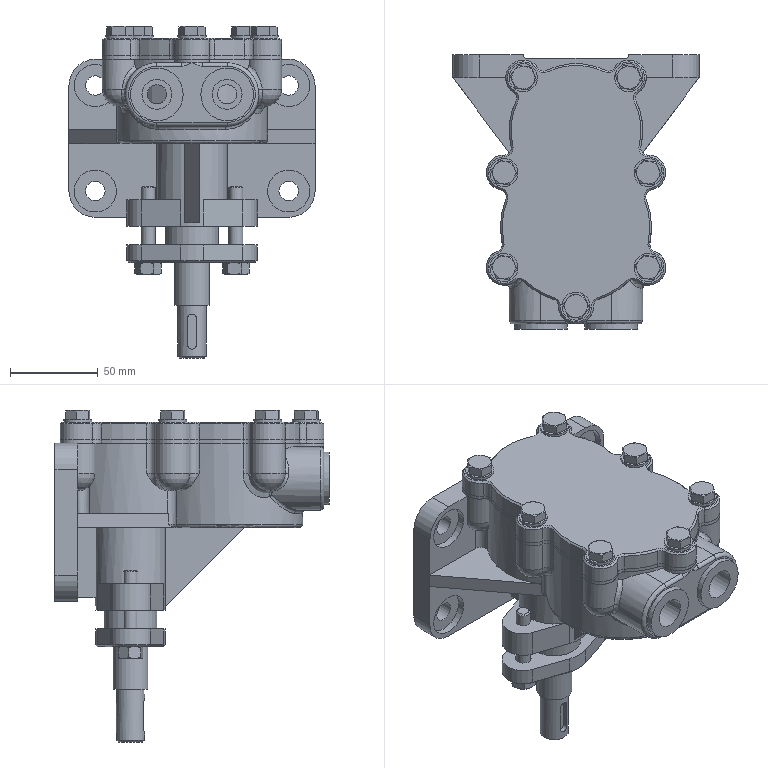Assembly | NX | mm | 27 component files | 32 solids | 522 faces | box 140 x 156 x 188.9 mm | volume 814585 mm3 | cylinder 197 | plane 188 | cone 81 | other 21 | torus 17 | spline 12 | sphere 6 | commonest cylinder face diameters 8 x58 20 x26 10 x14 86 x11 16 x9 30 x9 25 x9 76 x8
Bill of materials:
unnamed part 1 | 2 |  | Hexagonal nut-like prism with a central plain cylindrical through-bore and chamfered corners on both faces.
unnamed part 2 | 2 |  | Plain solid cylindrical rod or pin with small chamfers at both ends.
unnamed part 3 | 1 |  | Thin flat gasket-like plate with a figure-eight opening made of two overlapping circles, and seven rounded perimeter lugs, each with a through-hole.
unnamed part 4 | 1 |  | Solid flat plate with a lobed outline formed by two merged circles, and seven rounded lugs with through-holes around the edge. It looks like a cover plate.
unnamed part 5 | 7 |  | Hex-head bolt-like part: a hexagonal head with a chamfered top, on a plain cylindrical shank with a chamfered tip.
unnamed part 6 | 1 |  | Stepped cylindrical shaft with a thin disk-shaped collar near one end. A smaller pin sits above the collar, offset from the main axis. The opposite end steps down to a smaller diameter with a slot or flat.
unnamed part 7 | 1 |  | Thin-walled cylindrical tube or sleeve with plain ends and a small axial groove along the bore.
unnamed part 8 | 1 |  | Short solid cylinder with one radial through-hole across its diameter.
unnamed part 9 | 1 |  | Thick annular ring or bushing with a central through-bore and large chamfers on the outer edges at both ends.
unnamed part 10 | 7 |  | Complex housing-like body. It has a double-bore cavity shaped like a figure eight, surrounded by a flange with seven bolt holes, and is joined at right angles to a rectangular mounting plate with four corner holes. It also has cylindrical bosses or ports and a triangular stiffening rib.
unnamed part 11 | 1 |  | Solid cylindrical pin with chamfered ends, five shallow evenly spaced circumferential grooves along most of its length, and a radial through-hole near one end.
unnamed part 12 | 1 |  | Flat circular washer-like ring with a plain central hole and uniform thickness.
unnamed part 13 | 1 |  | Two-hole flanged cylindrical boss: a flat diamond/oval-shaped flange plate with rounded lobes, a through hole in each lobe, and a central raised cylindrical hub with a through bore.
Mates:
1. parallel | 6_disk 1 face | 1_pump_body 1 face
2. concentric | 2_side_cover 1 edge | 5_gasket 1 edge
3. concentric | 2_side_cover 1 edge | 5_gasket 1 edge
4. touch align | 6_disk 1 face | 11_plunger 1 face
5. touch align | 10_crankshaft 1 face | 1_pump_body 1 face
6. touch align | 10_crankshaft 1 face | 11_plunger 1 face
7. touch align | 10_crankshaft 1 face | 1_pump_body 1 face
8. concentric | packing 1 edge | 7_bushing 1
9. touch align | 9_packing_gland 1 face | 1_pump_body 1 face
10. concentric | 4_washer_8 7 edge | 2_side_cover 1 edge
11. concentric | 4_washer_8 5 edge | 2_side_cover 1 edge
12. concentric | 4_washer_8 4 edge | 2_side_cover 1 edge
13. concentric | 4_washer_8 6 edge | 2_side_cover 1 edge
14. concentric | 4_washer_8 1 edge | 2_side_cover 1 edge
15. concentric | 4_washer_8 2 edge | 2_side_cover 1 edge
16. concentric | 4_washer_8 3 edge | 2_side_cover 1 edge
17. concentric | 13_nut 2 | 9_packing_gland 1 edge
18. concentric | 12_stud 1 | 13_nut 2
19. parallel | 1_pump_body 1 face | assembly datumplane
20. concentric | 13_nut 1 arc | 9_packing_gland 1 edge
21. concentric | 13_nut 2 edge | 9_packing_gland 1 edge
22. concentric | 12_stud 1 arc | 13_nut 2 arc
23. concentric | 12_stud 2 arc | 13_nut 1 arc
24. concentric | 7_bushing 1 edge | packing 1 edge
25. touch align | packing 1 face | 9_packing_gland 1 face
26. touch align | packing 1 face | 9_packing_gland 1 face
27. touch align | 10_crankshaft 1 face | 7_bushing 1 face
28. concentric | 1_pump_body 1 edge | 6_disk 1 edge
29. concentric | 5_gasket 1 edge | 1_pump_body 1 edge
30. concentric | 3_bolt 7 edge | 4_washer_8 7 edge
31. concentric | 3_bolt 6 edge | 4_washer_8 5 edge
32. concentric | 3_bolt 1 edge | 4_washer_8 4 edge
33. concentric | 3_bolt 5 edge | 4_washer_8 3 edge
34. concentric | 3_bolt 4 edge | 4_washer_8 2 edge
35. concentric | 3_bolt 3 edge | 4_washer_8 1 edge
36. concentric | 3_bolt 2 edge | 4_washer_8 6 edge